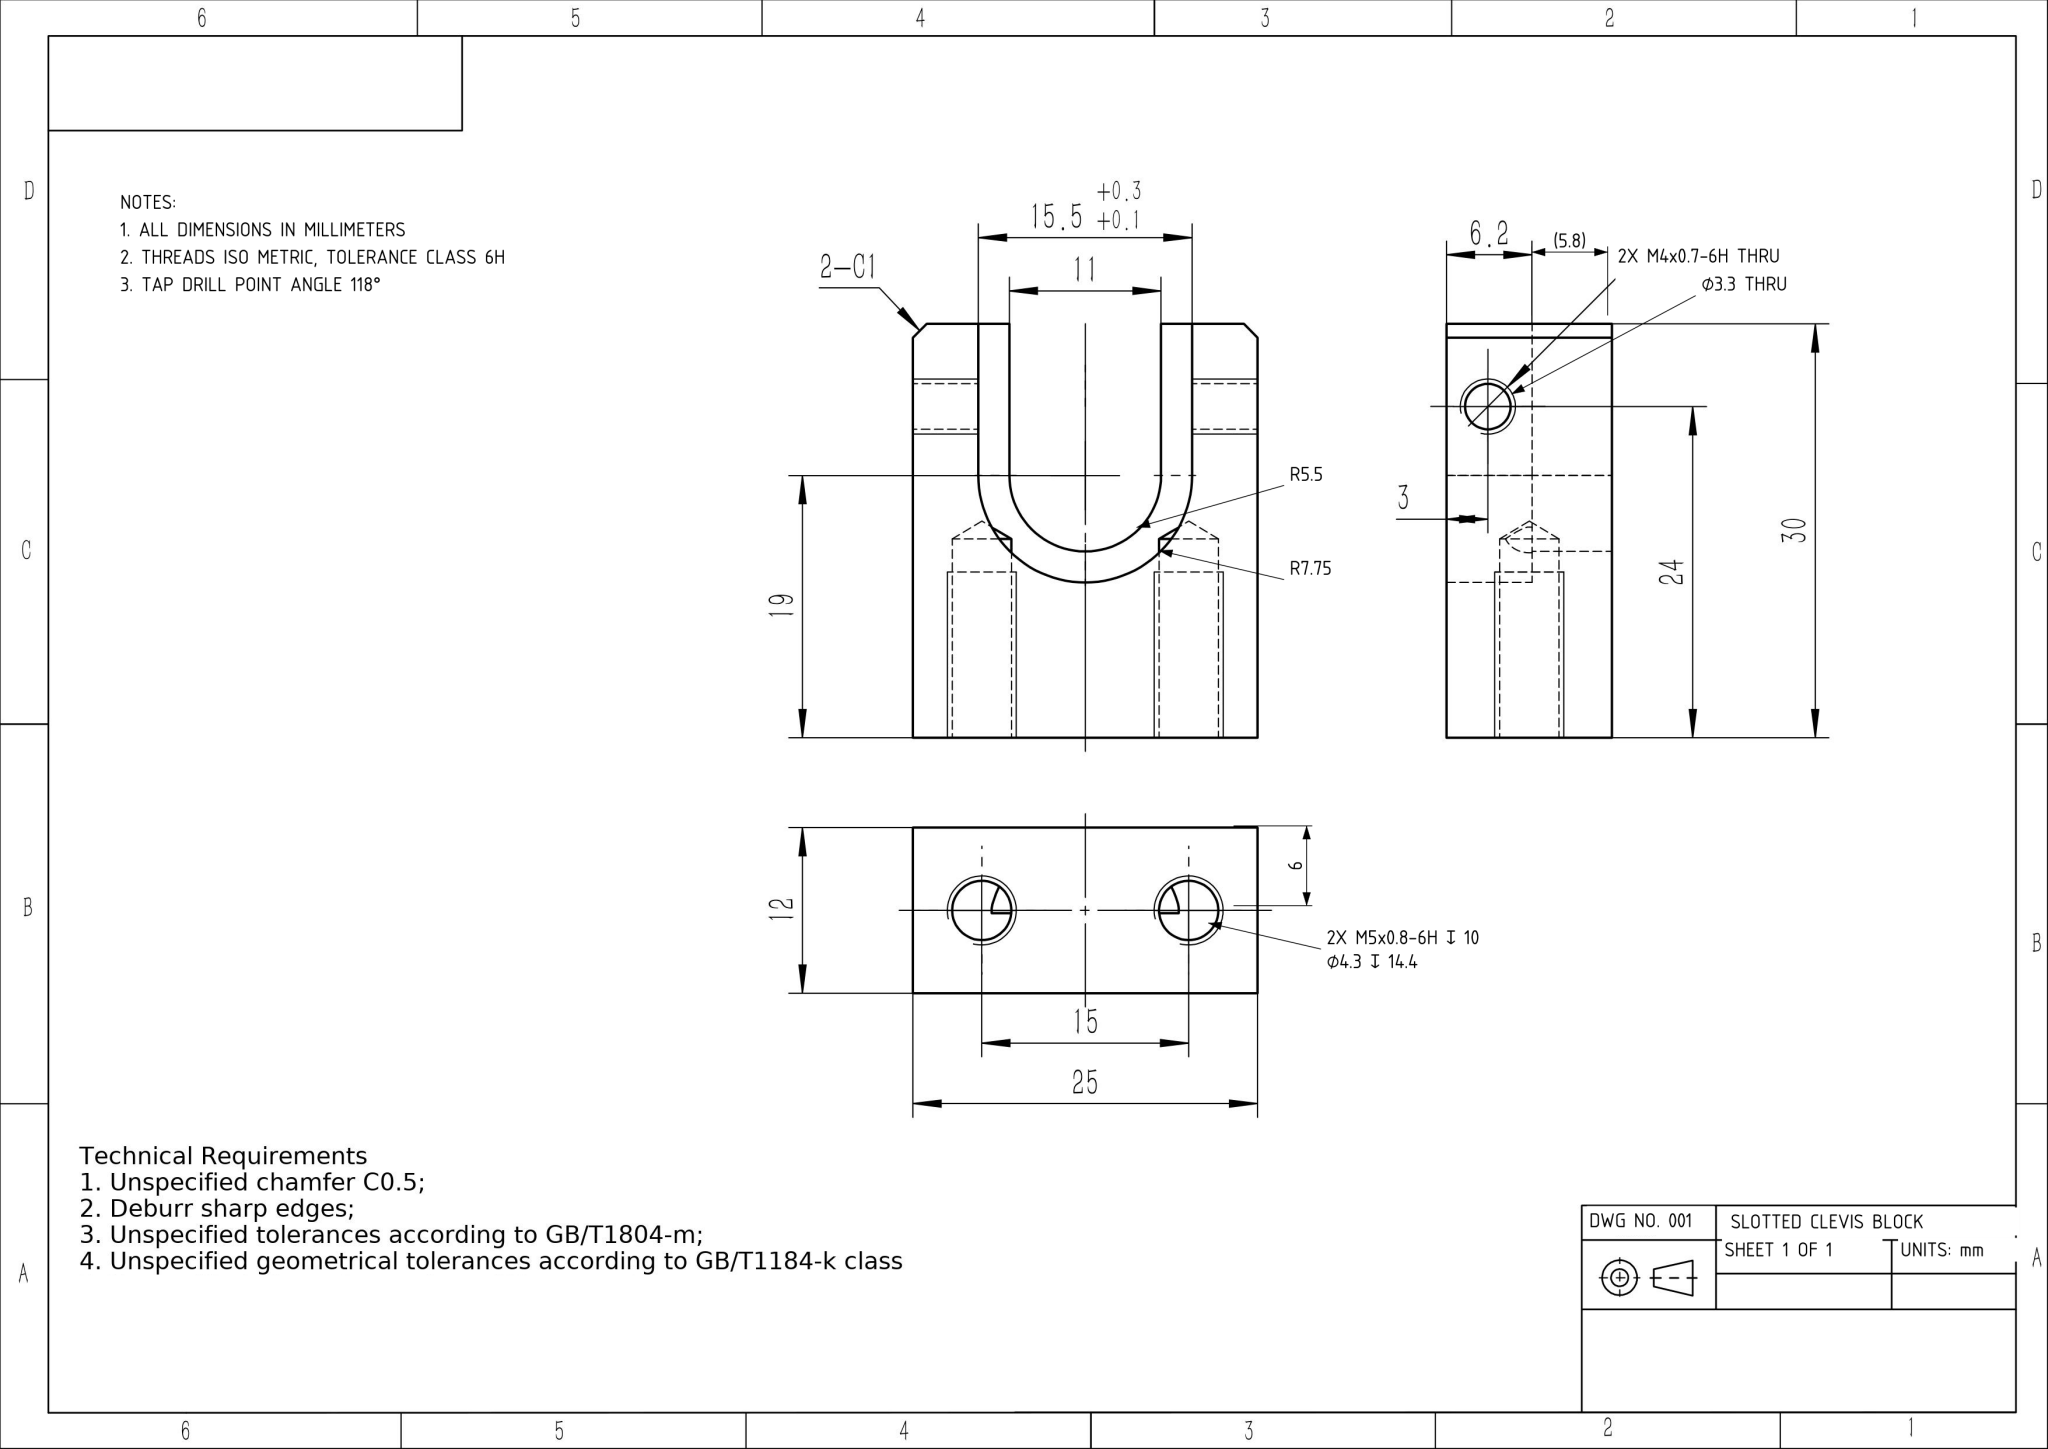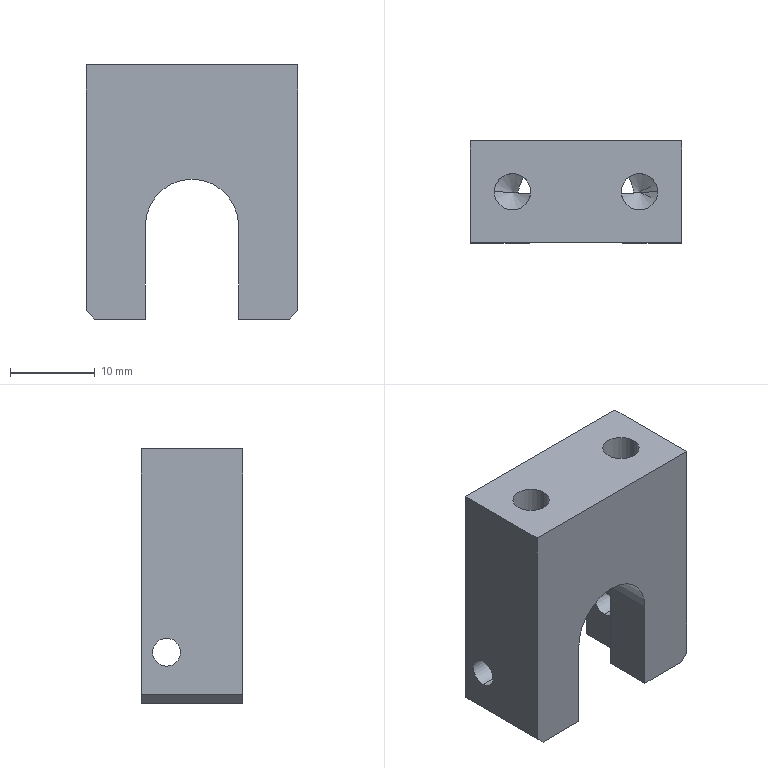Part | NX | mm | 1 solid | 30 faces | box 25 x 12 x 30 mm | volume 5859 mm3 | plane 14 | cylinder 12 | cone 4 | commonest cylinder face diameters 4.3 x4 3.3 x4 11 x2 15.5 x2